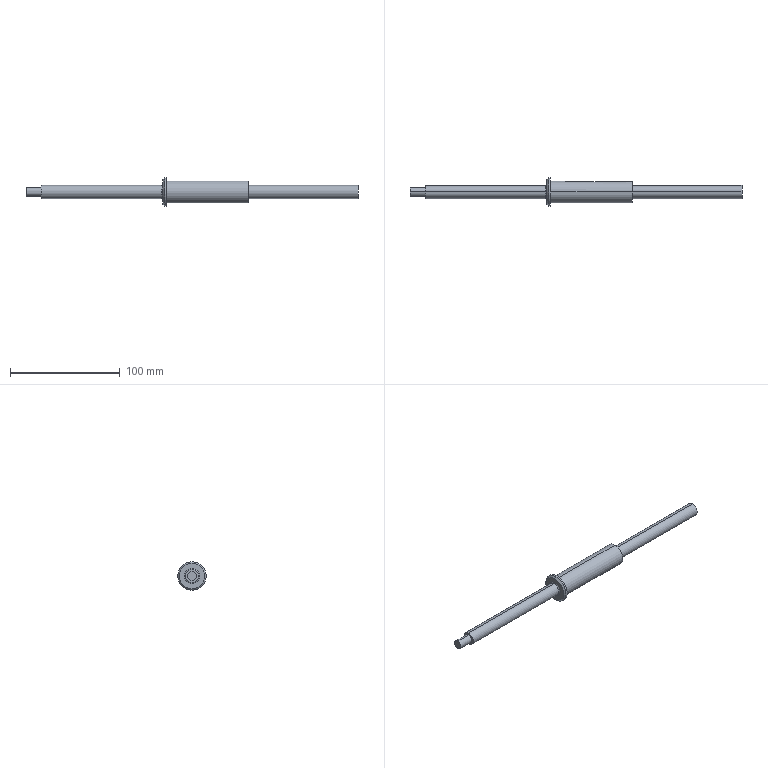Component | SolidWorks | ShortAxis(Modified)-1 | 1 solid | 28 faces | box 303 x 26 x 26 mm | volume 48394 mm3 | cylinder 11 | plane 9 | torus 6 | cone 2 | commonest cylinder face diameters 12 x4 8 x2 26 x2 20 x2 6 x1 | material AISI 1045 Steel, Cold Drawn
build123d program:
from build123d import *

# Parameters (mm, degrees)
FILLET3_R          = 0.5
FILLET6_R          = 1
CHAMFER1_SIZE      = 1.5
CUT_EXTRUDE1_DEPTH = 10


with BuildPart() as part:
    # Sketch1 → Revolve1 (revolve)
    with BuildSketch(Plane.XY, mode=Mode.PRIVATE) as revolve1_sk:
        Polygon((-152.849, 0), (-152.849, 6), (-52.849, 6), (-52.849, 10), (22.151, 10), (22.151, 13), (25.151, 13), (25.151, 6), (136.151, 6), (136.151, 4), (150.151, 4), (150.151, 0), align=None)
    revolve(revolve1_sk.sketch.rotate(Axis((-152.849, 0, 0), (1, 0, 0)), 90), axis=Axis((-152.849, 0, 0), (1, 0, 0)))

    # Fillet3
    fillet3_edges = [part.edges().sort_by_distance(p)[0] for p in [
        (22.151, 0, -10),
        (-52.849, 0, -6),
    ]]
    fillet(fillet3_edges, radius=FILLET3_R)

    # Fillet6
    fillet6_edges = [part.edges().sort_by_distance(p)[0] for p in [
        (25.151, 0, -6),
    ]]
    fillet(fillet6_edges, radius=FILLET6_R)

    # Chamfer1
    chamfer1_edges = [part.edges().sort_by_distance(p)[0] for p in [
        (25.151, 0, -13),
    ]]
    chamfer(chamfer1_edges, length=CHAMFER1_SIZE)

    # Sketch4 → Cut-Extrude1 (cut)
    with BuildSketch(Plane(origin=(0, 6.5, 0), x_dir=(1, 0, 0), z_dir=(0, 1, 0))):
        with BuildLine():
            Line((-63.443, -3), (7.151, -3))
            ThreePointArc((7.151, -3), (10.151, 0), (7.151, 3))
            Line((7.151, 3), (-63.443, 3))
            Line((-63.443, 3), (-63.443, -3))
        make_face()
    extrude(amount=CUT_EXTRUDE1_DEPTH, mode=Mode.SUBTRACT)


solid = part.part

# Placed as in the assembly
solid = solid.moved(Location((390.213, 15.116, 349), (-180, 0, 180)))
STEP:
#1=CARTESIAN_POINT('',(14.373,0.5951,14.193));
#2=VERTEX_POINT('',#1);
#3=CARTESIAN_POINT('',(14.373,0.5951,13.287));
#4=VERTEX_POINT('',#3);
#5=CARTESIAN_POINT('',(14.373,0.5951,13.74));
#6=DIRECTION('',(-1.,0.,0.));
#7=DIRECTION('',(0.,-0.,-1.));
#8=AXIS2_PLACEMENT_3D('',#5,#6,#7);
#9=CIRCLE('',#8,0.4528);
#10=EDGE_CURVE('',#2,#4,#9,.T.);
#11=ORIENTED_EDGE('',*,*,#10,.F.);
#12=CARTESIAN_POINT('',(14.432,0.5951,14.252));
#13=VERTEX_POINT('',#12);
#14=CARTESIAN_POINT('',(14.432,0.5951,14.252));
#15=DIRECTION('',(0.7071,0.,0.7071));
#16=VECTOR('',#15,39.37);
#17=LINE('',#14,#16);
#18=EDGE_CURVE('',#2,#13,#17,.T.);
#19=ORIENTED_EDGE('',*,*,#18,.T.);
#20=CARTESIAN_POINT('',(14.432,0.5951,13.228));
#21=VERTEX_POINT('',#20);
#22=CARTESIAN_POINT('',(14.432,0.5951,13.74));
#23=DIRECTION('',(1.,0.,0.));
#24=DIRECTION('',(0.,-0.,-1.));
#25=AXIS2_PLACEMENT_3D('',#22,#23,#24);
#26=CIRCLE('',#25,0.5118);
#27=EDGE_CURVE('',#21,#13,#26,.T.);
#28=ORIENTED_EDGE('',*,*,#27,.F.);
#29=CARTESIAN_POINT('',(14.432,0.5951,13.228));
#30=DIRECTION('',(0.7071,-0.,-0.7071));
#31=VECTOR('',#30,39.37);
#32=LINE('',#29,#31);
#33=EDGE_CURVE('',#4,#21,#32,.T.);
#34=ORIENTED_EDGE('',*,*,#33,.F.);
#35=EDGE_LOOP('',(#11,#19,#28,#34));
#36=FACE_OUTER_BOUND('',#35,.T.);
#37=CARTESIAN_POINT('',(14.432,0.5951,13.74));
#38=DIRECTION('',(1.,0.,0.));
#39=DIRECTION('',(0.,-0.,-1.));
#40=AXIS2_PLACEMENT_3D('',#37,#38,#39);
#41=CONICAL_SURFACE('',#40,0.5118,0.7854);
#42=ADVANCED_FACE('',(#36),#41,.T.);
#43=CARTESIAN_POINT('',(14.373,0.5951,14.016));
#44=VERTEX_POINT('',#43);
#45=CARTESIAN_POINT('',(14.373,0.5951,13.465));
#46=VERTEX_POINT('',#45);
#47=CARTESIAN_POINT('',(14.373,0.5951,13.74));
#48=DIRECTION('',(1.,0.,0.));
#49=DIRECTION('',(0.,0.,-1.));
#50=AXIS2_PLACEMENT_3D('',#47,#48,#49);
#51=CIRCLE('',#50,0.2756);
#52=EDGE_CURVE('',#44,#46,#51,.T.);
#53=ORIENTED_EDGE('',*,*,#52,.F.);
#54=CARTESIAN_POINT('',(14.333,0.5951,13.976));
#55=VERTEX_POINT('',#54);
#56=CARTESIAN_POINT('',(14.333,0.5951,14.016));
#57=DIRECTION('',(0.,1.,-0.));
#58=DIRECTION('',(0.,0.,1.));
#59=AXIS2_PLACEMENT_3D('',#56,#57,#58);
#60=CIRCLE('',#59,0.03937);
#61=EDGE_CURVE('',#44,#55,#60,.T.);
#62=ORIENTED_EDGE('',*,*,#61,.T.);
#63=CARTESIAN_POINT('',(14.333,0.5951,13.504));
#64=VERTEX_POINT('',#63);
#65=CARTESIAN_POINT('',(14.333,0.5951,13.74));
#66=DIRECTION('',(-1.,0.,0.));
#67=DIRECTION('',(0.,0.,-1.));
#68=AXIS2_PLACEMENT_3D('',#65,#66,#67);
#69=CIRCLE('',#68,0.2362);
#70=EDGE_CURVE('',#64,#55,#69,.T.);
#71=ORIENTED_EDGE('',*,*,#70,.F.);
#72=CARTESIAN_POINT('',(14.333,0.5951,13.465));
#73=DIRECTION('',(0.,-1.,0.));
#74=DIRECTION('',(0.,0.,-1.));
#75=AXIS2_PLACEMENT_3D('',#72,#73,#74);
#76=CIRCLE('',#75,0.03937);
#77=EDGE_CURVE('',#46,#64,#76,.T.);
#78=ORIENTED_EDGE('',*,*,#77,.F.);
#79=EDGE_LOOP('',(#53,#62,#71,#78));
#80=FACE_OUTER_BOUND('',#79,.T.);
#81=CARTESIAN_POINT('',(14.333,0.5951,13.74));
#82=DIRECTION('',(1.,0.,0.));
#83=DIRECTION('',(0.,-0.,-1.));
#84=AXIS2_PLACEMENT_3D('',#81,#82,#83);
#85=TOROIDAL_SURFACE('',#84,0.2756,0.03937);
#86=ADVANCED_FACE('',(#80),#85,.F.);
#87=CARTESIAN_POINT('',(17.443,0.5951,13.484));
#88=VERTEX_POINT('',#87);
#89=CARTESIAN_POINT('',(17.443,0.5951,13.996));
#90=VERTEX_POINT('',#89);
#91=CARTESIAN_POINT('',(17.443,0.5951,13.74));
#92=DIRECTION('',(-1.,0.,0.));
#93=DIRECTION('',(0.,0.,1.));
#94=AXIS2_PLACEMENT_3D('',#91,#92,#93);
#95=CIRCLE('',#94,0.2559);
#96=EDGE_CURVE('',#88,#90,#95,.T.);
#97=ORIENTED_EDGE('',*,*,#96,.F.);
#98=CARTESIAN_POINT('',(17.463,0.5951,13.504));
#99=VERTEX_POINT('',#98);
#100=CARTESIAN_POINT('',(17.463,0.5951,13.484));
#101=DIRECTION('',(0.,1.,0.));
#102=DIRECTION('',(0.,0.,1.));
#103=AXIS2_PLACEMENT_3D('',#100,#101,#102);
#104=CIRCLE('',#103,0.01969);
#105=EDGE_CURVE('',#88,#99,#104,.T.);
#106=ORIENTED_EDGE('',*,*,#105,.T.);
#107=CARTESIAN_POINT('',(17.463,0.5951,13.976));
#108=VERTEX_POINT('',#107);
#109=CARTESIAN_POINT('',(17.463,0.5951,13.74));
#110=DIRECTION('',(1.,0.,0.));
#111=DIRECTION('',(0.,0.,1.));
#112=AXIS2_PLACEMENT_3D('',#109,#110,#111);
#113=CIRCLE('',#112,0.2362);
#114=EDGE_CURVE('',#108,#99,#113,.T.);
#115=ORIENTED_EDGE('',*,*,#114,.F.);
#116=CARTESIAN_POINT('',(17.463,0.5951,13.996));
#117=DIRECTION('',(0.,-1.,0.));
#118=DIRECTION('',(0.,0.,-1.));
#119=AXIS2_PLACEMENT_3D('',#116,#117,#118);
#120=CIRCLE('',#119,0.01969);
#121=EDGE_CURVE('',#90,#108,#120,.T.);
#122=ORIENTED_EDGE('',*,*,#121,.F.);
#123=EDGE_LOOP('',(#97,#106,#115,#122));
#124=FACE_OUTER_BOUND('',#123,.T.);
#125=CARTESIAN_POINT('',(17.463,0.5951,13.74));
#126=DIRECTION('',(-1.,0.,0.));
#127=DIRECTION('',(0.,0.,1.));
#128=AXIS2_PLACEMENT_3D('',#125,#126,#127);
#129=TOROIDAL_SURFACE('',#128,0.2559,0.01969);
#130=ADVANCED_FACE('',(#124),#129,.F.);
#131=CARTESIAN_POINT('',(14.491,0.5951,13.327));
#132=VERTEX_POINT('',#131);
#133=CARTESIAN_POINT('',(14.491,0.5951,14.154));
#134=VERTEX_POINT('',#133);
#135=CARTESIAN_POINT('',(14.491,0.5951,13.74));
#136=DIRECTION('',(-1.,0.,0.));
#137=DIRECTION('',(0.,0.,1.));
#138=AXIS2_PLACEMENT_3D('',#135,#136,#137);
#139=CIRCLE('',#138,0.4134);
#140=EDGE_CURVE('',#132,#134,#139,.T.);
#141=ORIENTED_EDGE('',*,*,#140,.F.);
#142=CARTESIAN_POINT('',(14.51,0.5951,13.346));
#143=VERTEX_POINT('',#142);
#144=CARTESIAN_POINT('',(14.51,0.5951,13.327));
#145=DIRECTION('',(0.,1.,0.));
#146=DIRECTION('',(0.,0.,1.));
#147=AXIS2_PLACEMENT_3D('',#144,#145,#146);
#148=CIRCLE('',#147,0.01969);
#149=EDGE_CURVE('',#132,#143,#148,.T.);
#150=ORIENTED_EDGE('',*,*,#149,.T.);
#151=CARTESIAN_POINT('',(14.51,0.5951,14.134));
#152=VERTEX_POINT('',#151);
#153=CARTESIAN_POINT('',(14.51,0.5951,13.74));
#154=DIRECTION('',(1.,0.,0.));
#155=DIRECTION('',(0.,0.,1.));
#156=AXIS2_PLACEMENT_3D('',#153,#154,#155);
#157=CIRCLE('',#156,0.3937);
#158=EDGE_CURVE('',#152,#143,#157,.T.);
#159=ORIENTED_EDGE('',*,*,#158,.F.);
#160=CARTESIAN_POINT('',(14.51,0.5951,14.154));
#161=DIRECTION('',(0.,-1.,0.));
#162=DIRECTION('',(0.,0.,-1.));
#163=AXIS2_PLACEMENT_3D('',#160,#161,#162);
#164=CIRCLE('',#163,0.01969);
#165=EDGE_CURVE('',#134,#152,#164,.T.);
#166=ORIENTED_EDGE('',*,*,#165,.F.);
#167=EDGE_LOOP('',(#141,#150,#159,#166));
#168=FACE_OUTER_BOUND('',#167,.T.);
#169=CARTESIAN_POINT('',(14.51,0.5951,13.74));
#170=DIRECTION('',(-1.,0.,0.));
#171=DIRECTION('',(0.,0.,1.));
#172=AXIS2_PLACEMENT_3D('',#169,#170,#171);
#173=TOROIDAL_SURFACE('',#172,0.4134,0.01969);
#174=ADVANCED_FACE('',(#168),#173,.F.);
#175=CARTESIAN_POINT('',(9.451,0.5951,13.583));
#176=VERTEX_POINT('',#175);
#177=CARTESIAN_POINT('',(9.451,0.5951,13.898));
#178=VERTEX_POINT('',#177);
#179=CARTESIAN_POINT('',(9.451,0.5951,13.74));
#180=DIRECTION('',(1.,0.,0.));
#181=DIRECTION('',(0.,0.,-1.));
#182=AXIS2_PLACEMENT_3D('',#179,#180,#181);
#183=CIRCLE('',#182,0.1575);
#184=EDGE_CURVE('',#176,#178,#183,.T.);
#185=ORIENTED_EDGE('',*,*,#184,.T.);
#186=CARTESIAN_POINT('',(10.002,0.5951,13.898));
#187=VERTEX_POINT('',#186);
#188=CARTESIAN_POINT('',(21.38,0.5951,13.898));
#189=DIRECTION('',(1.,0.,0.));
#190=VECTOR('',#189,39.37);
#191=LINE('',#188,#190);
#192=EDGE_CURVE('',#178,#187,#191,.T.);
#193=ORIENTED_EDGE('',*,*,#192,.T.);
#194=CARTESIAN_POINT('',(10.002,0.5951,13.583));
#195=VERTEX_POINT('',#194);
#196=CARTESIAN_POINT('',(10.002,0.5951,13.74));
#197=DIRECTION('',(1.,0.,0.));
#198=DIRECTION('',(0.,0.,-1.));
#199=AXIS2_PLACEMENT_3D('',#196,#197,#198);
#200=CIRCLE('',#199,0.1575);
#201=EDGE_CURVE('',#195,#187,#200,.T.);
#202=ORIENTED_EDGE('',*,*,#201,.F.);
#203=CARTESIAN_POINT('',(21.38,0.5951,13.583));
#204=DIRECTION('',(1.,0.,0.));
#205=VECTOR('',#204,39.37);
#206=LINE('',#203,#205);
#207=EDGE_CURVE('',#176,#195,#206,.T.);
#208=ORIENTED_EDGE('',*,*,#207,.F.);
#209=EDGE_LOOP('',(#185,#193,#202,#208));
#210=FACE_OUTER_BOUND('',#209,.T.);
#211=CARTESIAN_POINT('',(21.38,0.5951,13.74));
#212=DIRECTION('',(1.,0.,0.));
#213=DIRECTION('',(0.,0.,-1.));
#214=AXIS2_PLACEMENT_3D('',#211,#212,#213);
#215=CYLINDRICAL_SURFACE('',#214,0.1575);
#216=ADVANCED_FACE('',(#210),#215,.T.);
#217=CARTESIAN_POINT('',(10.002,0.5951,13.504));
#218=VERTEX_POINT('',#217);
#219=CARTESIAN_POINT('',(10.002,0.5951,13.976));
#220=VERTEX_POINT('',#219);
#221=CARTESIAN_POINT('',(10.002,0.5951,13.74));
#222=DIRECTION('',(1.,0.,0.));
#223=DIRECTION('',(0.,0.,-1.));
#224=AXIS2_PLACEMENT_3D('',#221,#222,#223);
#225=CIRCLE('',#224,0.2362);
#226=EDGE_CURVE('',#218,#220,#225,.T.);
#227=ORIENTED_EDGE('',*,*,#226,.T.);
#228=CARTESIAN_POINT('',(21.38,0.5951,13.976));
#229=DIRECTION('',(1.,0.,0.));
#230=VECTOR('',#229,39.37);
#231=LINE('',#228,#230);
#232=EDGE_CURVE('',#220,#55,#231,.T.);
#233=ORIENTED_EDGE('',*,*,#232,.T.);
#234=CARTESIAN_POINT('',(14.333,0.5951,13.74));
#235=DIRECTION('',(-1.,0.,0.));
#236=DIRECTION('',(0.,0.,-1.));
#237=AXIS2_PLACEMENT_3D('',#234,#235,#236);
#238=CIRCLE('',#237,0.2362);
#239=EDGE_CURVE('',#55,#64,#238,.T.);
#240=ORIENTED_EDGE('',*,*,#239,.T.);
#241=CARTESIAN_POINT('',(21.38,0.5951,13.504));
#242=DIRECTION('',(1.,0.,0.));
#243=VECTOR('',#242,39.37);
#244=LINE('',#241,#243);
#245=EDGE_CURVE('',#218,#64,#244,.T.);
#246=ORIENTED_EDGE('',*,*,#245,.F.);
#247=EDGE_LOOP('',(#227,#233,#240,#246));
#248=FACE_OUTER_BOUND('',#247,.T.);
#249=CARTESIAN_POINT('',(21.38,0.5951,13.74));
#250=DIRECTION('',(1.,0.,0.));
#251=DIRECTION('',(0.,0.,-1.));
#252=AXIS2_PLACEMENT_3D('',#249,#250,#251);
#253=CYLINDRICAL_SURFACE('',#252,0.2362);
#254=ADVANCED_FACE('',(#248),#253,.T.);
#255=ORIENTED_EDGE('',*,*,#27,.T.);
#256=CARTESIAN_POINT('',(14.491,0.5951,14.252));
#257=VERTEX_POINT('',#256);
#258=CARTESIAN_POINT('',(21.38,0.5951,14.252));
#259=DIRECTION('',(1.,0.,0.));
#260=VECTOR('',#259,39.37);
#261=LINE('',#258,#260);
#262=EDGE_CURVE('',#13,#257,#261,.T.);
#263=ORIENTED_EDGE('',*,*,#262,.T.);
#264=CARTESIAN_POINT('',(14.491,0.5951,13.228));
#265=VERTEX_POINT('',#264);
#266=CARTESIAN_POINT('',(14.491,0.5951,13.74));
#267=DIRECTION('',(1.,0.,0.));
#268=DIRECTION('',(0.,-0.,-1.));
#269=AXIS2_PLACEMENT_3D('',#266,#267,#268);
#270=CIRCLE('',#269,0.5118);
#271=EDGE_CURVE('',#265,#257,#270,.T.);
#272=ORIENTED_EDGE('',*,*,#271,.F.);
#273=CARTESIAN_POINT('',(21.38,0.5951,13.228));
#274=DIRECTION('',(1.,0.,0.));
#275=VECTOR('',#274,39.37);
#276=LINE('',#273,#275);
#277=EDGE_CURVE('',#21,#265,#276,.T.);
#278=ORIENTED_EDGE('',*,*,#277,.F.);
#279=EDGE_LOOP('',(#255,#263,#272,#278));
#280=FACE_OUTER_BOUND('',#279,.T.);
#281=CARTESIAN_POINT('',(21.38,0.5951,13.74));
#282=DIRECTION('',(1.,0.,0.));
#283=DIRECTION('',(0.,-0.,-1.));
#284=AXIS2_PLACEMENT_3D('',#281,#282,#283);
#285=CYLINDRICAL_SURFACE('',#284,0.5118);
#286=ADVANCED_FACE('',(#280),#285,.T.);
#287=CARTESIAN_POINT('',(17.463,0.5951,13.74));
#288=DIRECTION('',(1.,0.,0.));
#289=DIRECTION('',(0.,0.,1.));
#290=AXIS2_PLACEMENT_3D('',#287,#288,#289);
#291=CIRCLE('',#290,0.2362);
#292=EDGE_CURVE('',#99,#108,#291,.T.);
#293=ORIENTED_EDGE('',*,*,#292,.T.);
#294=CARTESIAN_POINT('',(21.38,0.5951,13.976));
#295=VERTEX_POINT('',#294);
#296=CARTESIAN_POINT('',(21.38,0.5951,13.976));
#297=DIRECTION('',(1.,0.,0.));
#298=VECTOR('',#297,39.37);
#299=LINE('',#296,#298);
#300=EDGE_CURVE('',#108,#295,#299,.T.);
#301=ORIENTED_EDGE('',*,*,#300,.T.);
#302=CARTESIAN_POINT('',(21.38,0.5951,13.504));
#303=VERTEX_POINT('',#302);
#304=CARTESIAN_POINT('',(21.38,0.5951,13.74));
#305=DIRECTION('',(1.,0.,0.));
#306=DIRECTION('',(0.,0.,-1.));
#307=AXIS2_PLACEMENT_3D('',#304,#305,#306);
#308=CIRCLE('',#307,0.2362);
#309=EDGE_CURVE('',#303,#295,#308,.T.);
#310=ORIENTED_EDGE('',*,*,#309,.F.);
#311=CARTESIAN_POINT('',(21.38,0.5951,13.504));
#312=DIRECTION('',(1.,0.,0.));
#313=VECTOR('',#312,39.37);
#314=LINE('',#311,#313);
#315=EDGE_CURVE('',#99,#303,#314,.T.);
#316=ORIENTED_EDGE('',*,*,#315,.F.);
#317=EDGE_LOOP('',(#293,#301,#310,#316));
#318=FACE_OUTER_BOUND('',#317,.T.);
#319=CARTESIAN_POINT('',(21.38,0.5951,13.74));
#320=DIRECTION('',(1.,0.,0.));
#321=DIRECTION('',(0.,0.,-1.));
#322=AXIS2_PLACEMENT_3D('',#319,#320,#321);
#323=CYLINDRICAL_SURFACE('',#322,0.2362);
#324=ADVANCED_FACE('',(#318),#323,.T.);
#325=CARTESIAN_POINT('',(14.51,0.5951,13.74));
#326=DIRECTION('',(1.,0.,0.));
#327=DIRECTION('',(0.,0.,1.));
#328=AXIS2_PLACEMENT_3D('',#325,#326,#327);
#329=CIRCLE('',#328,0.3937);
#330=EDGE_CURVE('',#143,#152,#329,.T.);
#331=ORIENTED_EDGE('',*,*,#330,.T.);
#332=CARTESIAN_POINT('',(17.443,0.5951,14.134));
#333=VERTEX_POINT('',#332);
#334=CARTESIAN_POINT('',(21.38,0.5951,14.134));
#335=DIRECTION('',(1.,0.,0.));
#336=VECTOR('',#335,39.37);
#337=LINE('',#334,#336);
#338=EDGE_CURVE('',#152,#333,#337,.T.);
#339=ORIENTED_EDGE('',*,*,#338,.T.);
#340=CARTESIAN_POINT('',(17.443,0.9707,13.858));
#341=VERTEX_POINT('',#340);
#342=CARTESIAN_POINT('',(17.443,0.5951,13.74));
#343=DIRECTION('',(1.,0.,0.));
#344=DIRECTION('',(0.,-0.,-1.));
#345=AXIS2_PLACEMENT_3D('',#342,#343,#344);
#346=CIRCLE('',#345,0.3937);
#347=EDGE_CURVE('',#341,#333,#346,.T.);
#348=ORIENTED_EDGE('',*,*,#347,.F.);
#349=CARTESIAN_POINT('',(15.081,0.9707,13.858));
#350=VERTEX_POINT('',#349);
#351=CARTESIAN_POINT('',(21.38,0.9707,13.858));
#352=DIRECTION('',(1.,0.,0.));
#353=VECTOR('',#352,39.37);
#354=LINE('',#351,#353);
#355=EDGE_CURVE('',#350,#341,#354,.T.);
#356=ORIENTED_EDGE('',*,*,#355,.F.);
#357=CARTESIAN_POINT('',(15.081,0.9707,13.622));
#358=VERTEX_POINT('',#357);
#359=CARTESIAN_POINT('',(15.081,0.9707,13.622));
#360=CARTESIAN_POINT('',(15.073,0.9707,13.622));
#361=CARTESIAN_POINT('',(15.066,0.9709,13.623));
#362=CARTESIAN_POINT('',(15.05,0.9718,13.626));
#363=CARTESIAN_POINT('',(15.043,0.9725,13.628));
#364=CARTESIAN_POINT('',(15.029,0.9743,13.634));
#365=CARTESIAN_POINT('',(15.022,0.9753,13.638));
#366=CARTESIAN_POINT('',(15.009,0.9775,13.646));
#367=CARTESIAN_POINT('',(15.003,0.9787,13.651));
#368=CARTESIAN_POINT('',(14.987,0.9822,13.667));
#369=CARTESIAN_POINT('',(14.978,0.9845,13.681));
#370=CARTESIAN_POINT('',(14.969,0.987,13.702));
#371=CARTESIAN_POINT('',(14.967,0.9877,13.709));
#372=CARTESIAN_POINT('',(14.964,0.9886,13.725));
#373=CARTESIAN_POINT('',(14.963,0.9888,13.732));
#374=CARTESIAN_POINT('',(14.963,0.9888,13.748));
#375=CARTESIAN_POINT('',(14.964,0.9886,13.756));
#376=CARTESIAN_POINT('',(14.967,0.9877,13.771));
#377=CARTESIAN_POINT('',(14.969,0.987,13.778));
#378=CARTESIAN_POINT('',(14.975,0.9854,13.793));
#379=CARTESIAN_POINT('',(14.979,0.9844,13.799));
#380=CARTESIAN_POINT('',(14.987,0.9822,13.812));
#381=CARTESIAN_POINT('',(14.992,0.981,13.818));
#382=CARTESIAN_POINT('',(15.003,0.9787,13.829));
#383=CARTESIAN_POINT('',(15.009,0.9775,13.834));
#384=CARTESIAN_POINT('',(15.022,0.9753,13.843));
#385=CARTESIAN_POINT('',(15.029,0.9743,13.846));
#386=CARTESIAN_POINT('',(15.043,0.9726,13.852));
#387=CARTESIAN_POINT('',(15.05,0.9719,13.854));
#388=CARTESIAN_POINT('',(15.065,0.9709,13.857));
#389=CARTESIAN_POINT('',(15.073,0.9707,13.858));
#390=CARTESIAN_POINT('',(15.081,0.9707,13.858));
#391=B_SPLINE_CURVE_WITH_KNOTS('',3,(#359,#360,#361,#362,#363,#364,#365,#366,#367,#368,#369,#370,#371,#372,#373,#374,#375,#376,#377,#378,#379,#380,#381,#382,#383,#384,#385,#386,#387,#388,#389,#390),.UNSPECIFIED.,.F.,.F.,(4,2,2,2,2,2,2,2,2,2,2,2,2,2,2,4),(0.,0.0005894,0.001179,0.001768,0.002358,0.003536,0.004126,0.004715,0.005305,0.005894,0.006484,0.007073,0.007662,0.008252,0.008841,0.009431),.UNSPECIFIED.);
#392=EDGE_CURVE('',#358,#350,#391,.T.);
#393=ORIENTED_EDGE('',*,*,#392,.F.);
#394=CARTESIAN_POINT('',(17.443,0.9707,13.622));
#395=VERTEX_POINT('',#394);
#396=CARTESIAN_POINT('',(21.38,0.9707,13.622));
#397=DIRECTION('',(-1.,0.,0.));
#398=VECTOR('',#397,39.37);
#399=LINE('',#396,#398);
#400=EDGE_CURVE('',#395,#358,#399,.T.);
#401=ORIENTED_EDGE('',*,*,#400,.F.);
#402=CARTESIAN_POINT('',(17.443,0.5951,13.346));
#403=VERTEX_POINT('',#402);
#404=CARTESIAN_POINT('',(17.443,0.5951,13.74));
#405=DIRECTION('',(1.,0.,0.));
#406=DIRECTION('',(0.,-0.,-1.));
#407=AXIS2_PLACEMENT_3D('',#404,#405,#406);
#408=CIRCLE('',#407,0.3937);
#409=EDGE_CURVE('',#403,#395,#408,.T.);
#410=ORIENTED_EDGE('',*,*,#409,.F.);
#411=CARTESIAN_POINT('',(21.38,0.5951,13.346));
#412=DIRECTION('',(1.,0.,0.));
#413=VECTOR('',#412,39.37);
#414=LINE('',#411,#413);
#415=EDGE_CURVE('',#143,#403,#414,.T.);
#416=ORIENTED_EDGE('',*,*,#415,.F.);
#417=EDGE_LOOP('',(#331,#339,#348,#356,#393,#401,#410,#416));
#418=FACE_OUTER_BOUND('',#417,.T.);
#419=CARTESIAN_POINT('',(21.38,0.5951,13.74));
#420=DIRECTION('',(1.,0.,0.));
#421=DIRECTION('',(0.,-0.,-1.));
#422=AXIS2_PLACEMENT_3D('',#419,#420,#421);
#423=CYLINDRICAL_SURFACE('',#422,0.3937);
#424=ADVANCED_FACE('',(#418),#423,.T.);
#425=CARTESIAN_POINT('',(17.443,0.851,13.858));
#426=VERTEX_POINT('',#425);
#427=CARTESIAN_POINT('',(17.443,0.8313,13.858));
#428=DIRECTION('',(0.,-1.,0.));
#429=VECTOR('',#428,39.37);
#430=LINE('',#427,#429);
#431=EDGE_CURVE('',#341,#426,#430,.T.);
#432=ORIENTED_EDGE('',*,*,#431,.F.);
#433=ORIENTED_EDGE('',*,*,#347,.T.);
#434=CARTESIAN_POINT('',(17.443,0.5951,13.74));
#435=DIRECTION('',(1.,0.,0.));
#436=DIRECTION('',(0.,-0.,-1.));
#437=AXIS2_PLACEMENT_3D('',#434,#435,#436);
#438=CIRCLE('',#437,0.3937);
#439=EDGE_CURVE('',#333,#403,#438,.T.);
#440=ORIENTED_EDGE('',*,*,#439,.T.);
#441=ORIENTED_EDGE('',*,*,#409,.T.);
#442=CARTESIAN_POINT('',(17.443,0.851,13.622));
#443=VERTEX_POINT('',#442);
#444=CARTESIAN_POINT('',(17.443,0.8313,13.622));
#445=DIRECTION('',(0.,1.,-0.));
#446=VECTOR('',#445,39.37);
#447=LINE('',#444,#446);
#448=EDGE_CURVE('',#443,#395,#447,.T.);
#449=ORIENTED_EDGE('',*,*,#448,.F.);
#450=CARTESIAN_POINT('',(17.443,0.851,13.74));
#451=VERTEX_POINT('',#450);
#452=CARTESIAN_POINT('',(17.443,0.851,13.74));
#453=DIRECTION('',(0.,-0.,-1.));
#454=VECTOR('',#453,39.37);
#455=LINE('',#452,#454);
#456=EDGE_CURVE('',#451,#443,#455,.T.);
#457=ORIENTED_EDGE('',*,*,#456,.F.);
#458=CARTESIAN_POINT('',(17.443,0.5951,13.74));
#459=DIRECTION('',(-1.,0.,0.));
#460=DIRECTION('',(0.,0.,1.));
#461=AXIS2_PLACEMENT_3D('',#458,#459,#460);
#462=CIRCLE('',#461,0.2559);
#463=EDGE_CURVE('',#451,#88,#462,.T.);
#464=ORIENTED_EDGE('',*,*,#463,.T.);
#465=ORIENTED_EDGE('',*,*,#96,.T.);
#466=CARTESIAN_POINT('',(17.443,0.5951,13.74));
#467=DIRECTION('',(-1.,0.,0.));
#468=DIRECTION('',(0.,0.,1.));
#469=AXIS2_PLACEMENT_3D('',#466,#467,#468);
#470=CIRCLE('',#469,0.2559);
#471=EDGE_CURVE('',#90,#451,#470,.T.);
#472=ORIENTED_EDGE('',*,*,#471,.T.);
#473=CARTESIAN_POINT('',(17.443,0.851,13.74));
#474=DIRECTION('',(0.,-0.,-1.));
#475=VECTOR('',#474,39.37);
#476=LINE('',#473,#475);
#477=EDGE_CURVE('',#426,#451,#476,.T.);
#478=ORIENTED_EDGE('',*,*,#477,.F.);
#479=EDGE_LOOP('',(#432,#433,#440,#441,#449,#457,#464,#465,#472,#478));
#480=FACE_OUTER_BOUND('',#479,.T.);
#481=CARTESIAN_POINT('',(17.443,0.8313,13.74));
#482=DIRECTION('',(-1.,0.,0.));
#483=DIRECTION('',(0.,0.,1.));
#484=AXIS2_PLACEMENT_3D('',#481,#482,#483);
#485=PLANE('',#484);
#486=ADVANCED_FACE('',(#480),#485,.F.);
#487=ORIENTED_EDGE('',*,*,#338,.F.);
#488=ORIENTED_EDGE('',*,*,#158,.T.);
#489=ORIENTED_EDGE('',*,*,#415,.T.);
#490=ORIENTED_EDGE('',*,*,#439,.F.);
#491=EDGE_LOOP('',(#487,#488,#489,#490));
#492=FACE_OUTER_BOUND('',#491,.T.);
#493=CARTESIAN_POINT('',(21.38,0.5951,13.74));
#494=DIRECTION('',(1.,0.,0.));
#495=DIRECTION('',(0.,-0.,-1.));
#496=AXIS2_PLACEMENT_3D('',#493,#494,#495);
#497=CYLINDRICAL_SURFACE('',#496,0.3937);
#498=ADVANCED_FACE('',(#492),#497,.T.);
#499=ORIENTED_EDGE('',*,*,#309,.T.);
#500=CARTESIAN_POINT('',(21.38,0.5951,13.74));
#501=DIRECTION('',(1.,0.,0.));
#502=DIRECTION('',(0.,0.,-1.));
#503=AXIS2_PLACEMENT_3D('',#500,#501,#502);
#504=CIRCLE('',#503,0.2362);
#505=EDGE_CURVE('',#295,#303,#504,.T.);
#506=ORIENTED_EDGE('',*,*,#505,.T.);
#507=EDGE_LOOP('',(#499,#506));
#508=FACE_OUTER_BOUND('',#507,.T.);
#509=CARTESIAN_POINT('',(21.38,0.5951,13.74));
#510=DIRECTION('',(-1.,0.,0.));
#511=DIRECTION('',(0.,0.,1.));
#512=AXIS2_PLACEMENT_3D('',#509,#510,#511);
#513=PLANE('',#512);
#514=ADVANCED_FACE('',(#508),#513,.F.);
#515=ORIENTED_EDGE('',*,*,#300,.F.);
#516=ORIENTED_EDGE('',*,*,#114,.T.);
#517=ORIENTED_EDGE('',*,*,#315,.T.);
#518=ORIENTED_EDGE('',*,*,#505,.F.);
#519=EDGE_LOOP('',(#515,#516,#517,#518));
#520=FACE_OUTER_BOUND('',#519,.T.);
#521=CARTESIAN_POINT('',(21.38,0.5951,13.74));
#522=DIRECTION('',(1.,0.,0.));
#523=DIRECTION('',(0.,0.,-1.));
#524=AXIS2_PLACEMENT_3D('',#521,#522,#523);
#525=CYLINDRICAL_SURFACE('',#524,0.2362);
#526=ADVANCED_FACE('',(#520),#525,.T.);
#527=CARTESIAN_POINT('',(14.491,0.5951,13.74));
#528=DIRECTION('',(-1.,0.,0.));
#529=DIRECTION('',(0.,0.,1.));
#530=AXIS2_PLACEMENT_3D('',#527,#528,#529);
#531=CIRCLE('',#530,0.4134);
#532=EDGE_CURVE('',#134,#132,#531,.T.);
#533=ORIENTED_EDGE('',*,*,#532,.T.);
#534=ORIENTED_EDGE('',*,*,#140,.T.);
#535=EDGE_LOOP('',(#533,#534));
#536=FACE_BOUND('',#535,.T.);
#537=ORIENTED_EDGE('',*,*,#271,.T.);
#538=CARTESIAN_POINT('',(14.491,0.5951,13.74));
#539=DIRECTION('',(1.,0.,0.));
#540=DIRECTION('',(0.,-0.,-1.));
#541=AXIS2_PLACEMENT_3D('',#538,#539,#540);
#542=CIRCLE('',#541,0.5118);
#543=EDGE_CURVE('',#257,#265,#542,.T.);
#544=ORIENTED_EDGE('',*,*,#543,.T.);
#545=EDGE_LOOP('',(#537,#544));
#546=FACE_OUTER_BOUND('',#545,.T.);
#547=CARTESIAN_POINT('',(14.491,0.9888,13.74));
#548=DIRECTION('',(-1.,0.,0.));
#549=DIRECTION('',(0.,0.,1.));
#550=AXIS2_PLACEMENT_3D('',#547,#548,#549);
#551=PLANE('',#550);
#552=ADVANCED_FACE('',(#536,#546),#551,.F.);
#553=ORIENTED_EDGE('',*,*,#262,.F.);
#554=CARTESIAN_POINT('',(14.432,0.5951,13.74));
#555=DIRECTION('',(1.,0.,0.));
#556=DIRECTION('',(0.,-0.,-1.));
#557=AXIS2_PLACEMENT_3D('',#554,#555,#556);
#558=CIRCLE('',#557,0.5118);
#559=EDGE_CURVE('',#13,#21,#558,.T.);
#560=ORIENTED_EDGE('',*,*,#559,.T.);
#561=ORIENTED_EDGE('',*,*,#277,.T.);
#562=ORIENTED_EDGE('',*,*,#543,.F.);
#563=EDGE_LOOP('',(#553,#560,#561,#562));
#564=FACE_OUTER_BOUND('',#563,.T.);
#565=CARTESIAN_POINT('',(21.38,0.5951,13.74));
#566=DIRECTION('',(1.,0.,0.));
#567=DIRECTION('',(0.,-0.,-1.));
#568=AXIS2_PLACEMENT_3D('',#565,#566,#567);
#569=CYLINDRICAL_SURFACE('',#568,0.5118);
#570=ADVANCED_FACE('',(#564),#569,.T.);
#571=CARTESIAN_POINT('',(14.373,0.5951,13.74));
#572=DIRECTION('',(-1.,0.,0.));
#573=DIRECTION('',(0.,-0.,-1.));
#574=AXIS2_PLACEMENT_3D('',#571,#572,#573);
#575=CIRCLE('',#574,0.4528);
#576=EDGE_CURVE('',#4,#2,#575,.T.);
#577=ORIENTED_EDGE('',*,*,#576,.T.);
#578=ORIENTED_EDGE('',*,*,#10,.T.);
#579=EDGE_LOOP('',(#577,#578));
#580=FACE_OUTER_BOUND('',#579,.T.);
#581=CARTESIAN_POINT('',(14.373,0.5951,13.74));
#582=DIRECTION('',(1.,0.,0.));
#583=DIRECTION('',(0.,0.,-1.));
#584=AXIS2_PLACEMENT_3D('',#581,#582,#583);
#585=CIRCLE('',#584,0.2756);
#586=EDGE_CURVE('',#46,#44,#585,.T.);
#587=ORIENTED_EDGE('',*,*,#586,.T.);
#588=ORIENTED_EDGE('',*,*,#52,.T.);
#589=EDGE_LOOP('',(#587,#588));
#590=FACE_BOUND('',#589,.T.);
#591=CARTESIAN_POINT('',(14.373,1.107,13.74));
#592=DIRECTION('',(1.,0.,0.));
#593=DIRECTION('',(0.,-0.,-1.));
#594=AXIS2_PLACEMENT_3D('',#591,#592,#593);
#595=PLANE('',#594);
#596=ADVANCED_FACE('',(#580,#590),#595,.F.);
#597=ORIENTED_EDGE('',*,*,#232,.F.);
#598=CARTESIAN_POINT('',(10.002,0.5951,13.74));
#599=DIRECTION('',(1.,0.,0.));
#600=DIRECTION('',(0.,0.,-1.));
#601=AXIS2_PLACEMENT_3D('',#598,#599,#600);
#602=CIRCLE('',#601,0.2362);
#603=EDGE_CURVE('',#220,#218,#602,.T.);
#604=ORIENTED_EDGE('',*,*,#603,.T.);
#605=ORIENTED_EDGE('',*,*,#245,.T.);
#606=ORIENTED_EDGE('',*,*,#70,.T.);
#607=EDGE_LOOP('',(#597,#604,#605,#606));
#608=FACE_OUTER_BOUND('',#607,.T.);
#609=CARTESIAN_POINT('',(21.38,0.5951,13.74));
#610=DIRECTION('',(1.,0.,0.));
#611=DIRECTION('',(0.,0.,-1.));
#612=AXIS2_PLACEMENT_3D('',#609,#610,#611);
#613=CYLINDRICAL_SURFACE('',#612,0.2362);
#614=ADVANCED_FACE('',(#608),#613,.T.);
#615=ORIENTED_EDGE('',*,*,#226,.F.);
#616=ORIENTED_EDGE('',*,*,#603,.F.);
#617=EDGE_LOOP('',(#615,#616));
#618=FACE_OUTER_BOUND('',#617,.T.);
#619=ORIENTED_EDGE('',*,*,#201,.T.);
#620=CARTESIAN_POINT('',(10.002,0.5951,13.74));
#621=DIRECTION('',(1.,0.,0.));
#622=DIRECTION('',(0.,0.,-1.));
#623=AXIS2_PLACEMENT_3D('',#620,#621,#622);
#624=CIRCLE('',#623,0.1575);
#625=EDGE_CURVE('',#187,#195,#624,.T.);
#626=ORIENTED_EDGE('',*,*,#625,.T.);
#627=EDGE_LOOP('',(#619,#626));
#628=FACE_BOUND('',#627,.T.);
#629=CARTESIAN_POINT('',(10.002,0.8313,13.74));
#630=DIRECTION('',(1.,0.,0.));
#631=DIRECTION('',(0.,-0.,-1.));
#632=AXIS2_PLACEMENT_3D('',#629,#630,#631);
#633=PLANE('',#632);
#634=ADVANCED_FACE('',(#618,#628),#633,.F.);
#635=ORIENTED_EDGE('',*,*,#192,.F.);
#636=CARTESIAN_POINT('',(9.451,0.5951,13.74));
#637=DIRECTION('',(1.,0.,0.));
#638=DIRECTION('',(0.,0.,-1.));
#639=AXIS2_PLACEMENT_3D('',#636,#637,#638);
#640=CIRCLE('',#639,0.1575);
#641=EDGE_CURVE('',#178,#176,#640,.T.);
#642=ORIENTED_EDGE('',*,*,#641,.T.);
#643=ORIENTED_EDGE('',*,*,#207,.T.);
#644=ORIENTED_EDGE('',*,*,#625,.F.);
#645=EDGE_LOOP('',(#635,#642,#643,#644));
#646=FACE_OUTER_BOUND('',#645,.T.);
#647=CARTESIAN_POINT('',(21.38,0.5951,13.74));
#648=DIRECTION('',(1.,0.,0.));
#649=DIRECTION('',(0.,0.,-1.));
#650=AXIS2_PLACEMENT_3D('',#647,#648,#649);
#651=CYLINDRICAL_SURFACE('',#650,0.1575);
#652=ADVANCED_FACE('',(#646),#651,.T.);
#653=ORIENTED_EDGE('',*,*,#184,.F.);
#654=ORIENTED_EDGE('',*,*,#641,.F.);
#655=EDGE_LOOP('',(#653,#654));
#656=FACE_OUTER_BOUND('',#655,.T.);
#657=CARTESIAN_POINT('',(9.451,0.7526,13.74));
#658=DIRECTION('',(1.,0.,0.));
#659=DIRECTION('',(0.,-0.,-1.));
#660=AXIS2_PLACEMENT_3D('',#657,#658,#659);
#661=PLANE('',#660);
#662=ADVANCED_FACE('',(#656),#661,.F.);
#663=ORIENTED_EDGE('',*,*,#149,.F.);
#664=ORIENTED_EDGE('',*,*,#532,.F.);
#665=ORIENTED_EDGE('',*,*,#165,.T.);
#666=ORIENTED_EDGE('',*,*,#330,.F.);
#667=EDGE_LOOP('',(#663,#664,#665,#666));
#668=FACE_OUTER_BOUND('',#667,.T.);
#669=CARTESIAN_POINT('',(14.51,0.5951,13.74));
#670=DIRECTION('',(-1.,0.,0.));
#671=DIRECTION('',(0.,0.,1.));
#672=AXIS2_PLACEMENT_3D('',#669,#670,#671);
#673=TOROIDAL_SURFACE('',#672,0.4134,0.01969);
#674=ADVANCED_FACE('',(#668),#673,.F.);
#675=ORIENTED_EDGE('',*,*,#105,.F.);
#676=ORIENTED_EDGE('',*,*,#463,.F.);
#677=ORIENTED_EDGE('',*,*,#471,.F.);
#678=ORIENTED_EDGE('',*,*,#121,.T.);
#679=ORIENTED_EDGE('',*,*,#292,.F.);
#680=EDGE_LOOP('',(#675,#676,#677,#678,#679));
#681=FACE_OUTER_BOUND('',#680,.T.);
#682=CARTESIAN_POINT('',(17.463,0.5951,13.74));
#683=DIRECTION('',(-1.,0.,0.));
#684=DIRECTION('',(0.,0.,1.));
#685=AXIS2_PLACEMENT_3D('',#682,#683,#684);
#686=TOROIDAL_SURFACE('',#685,0.2559,0.01969);
#687=ADVANCED_FACE('',(#681),#686,.F.);
#688=ORIENTED_EDGE('',*,*,#61,.F.);
#689=ORIENTED_EDGE('',*,*,#586,.F.);
#690=ORIENTED_EDGE('',*,*,#77,.T.);
#691=ORIENTED_EDGE('',*,*,#239,.F.);
#692=EDGE_LOOP('',(#688,#689,#690,#691));
#693=FACE_OUTER_BOUND('',#692,.T.);
#694=CARTESIAN_POINT('',(14.333,0.5951,13.74));
#695=DIRECTION('',(1.,0.,0.));
#696=DIRECTION('',(0.,-0.,-1.));
#697=AXIS2_PLACEMENT_3D('',#694,#695,#696);
#698=TOROIDAL_SURFACE('',#697,0.2756,0.03937);
#699=ADVANCED_FACE('',(#693),#698,.F.);
#700=ORIENTED_EDGE('',*,*,#18,.F.);
#701=ORIENTED_EDGE('',*,*,#576,.F.);
#702=ORIENTED_EDGE('',*,*,#33,.T.);
#703=ORIENTED_EDGE('',*,*,#559,.F.);
#704=EDGE_LOOP('',(#700,#701,#702,#703));
#705=FACE_OUTER_BOUND('',#704,.T.);
#706=CARTESIAN_POINT('',(14.432,0.5951,13.74));
#707=DIRECTION('',(1.,0.,0.));
#708=DIRECTION('',(0.,-0.,-1.));
#709=AXIS2_PLACEMENT_3D('',#706,#707,#708);
#710=CONICAL_SURFACE('',#709,0.5118,0.7854);
#711=ADVANCED_FACE('',(#705),#710,.T.);
#712=ORIENTED_EDGE('',*,*,#392,.T.);
#713=CARTESIAN_POINT('',(15.081,0.851,13.858));
#714=VERTEX_POINT('',#713);
#715=CARTESIAN_POINT('',(15.081,1.245,13.858));
#716=DIRECTION('',(0.,-1.,0.));
#717=VECTOR('',#716,39.37);
#718=LINE('',#715,#717);
#719=EDGE_CURVE('',#350,#714,#718,.T.);
#720=ORIENTED_EDGE('',*,*,#719,.T.);
#721=CARTESIAN_POINT('',(15.081,0.851,13.622));
#722=VERTEX_POINT('',#721);
#723=CARTESIAN_POINT('',(15.081,0.851,13.74));
#724=DIRECTION('',(0.,1.,-0.));
#725=DIRECTION('',(0.,0.,-1.));
#726=AXIS2_PLACEMENT_3D('',#723,#724,#725);
#727=CIRCLE('',#726,0.1181);
#728=EDGE_CURVE('',#722,#714,#727,.T.);
#729=ORIENTED_EDGE('',*,*,#728,.F.);
#730=CARTESIAN_POINT('',(15.081,1.245,13.622));
#731=DIRECTION('',(0.,-1.,0.));
#732=VECTOR('',#731,39.37);
#733=LINE('',#730,#732);
#734=EDGE_CURVE('',#358,#722,#733,.T.);
#735=ORIENTED_EDGE('',*,*,#734,.F.);
#736=EDGE_LOOP('',(#712,#720,#729,#735));
#737=FACE_OUTER_BOUND('',#736,.T.);
#738=CARTESIAN_POINT('',(15.081,1.245,13.74));
#739=DIRECTION('',(0.,-1.,0.));
#740=DIRECTION('',(0.,0.,1.));
#741=AXIS2_PLACEMENT_3D('',#738,#739,#740);
#742=CYLINDRICAL_SURFACE('',#741,0.1181);
#743=ADVANCED_FACE('',(#737),#742,.F.);
#744=ORIENTED_EDGE('',*,*,#431,.T.);
#745=CARTESIAN_POINT('',(17.86,0.851,13.858));
#746=DIRECTION('',(1.,0.,0.));
#747=VECTOR('',#746,39.37);
#748=LINE('',#745,#747);
#749=EDGE_CURVE('',#714,#426,#748,.T.);
#750=ORIENTED_EDGE('',*,*,#749,.F.);
#751=ORIENTED_EDGE('',*,*,#719,.F.);
#752=ORIENTED_EDGE('',*,*,#355,.T.);
#753=EDGE_LOOP('',(#744,#750,#751,#752));
#754=FACE_OUTER_BOUND('',#753,.T.);
#755=CARTESIAN_POINT('',(17.86,1.245,13.858));
#756=DIRECTION('',(0.,-0.,-1.));
#757=DIRECTION('',(-1.,0.,0.));
#758=AXIS2_PLACEMENT_3D('',#755,#756,#757);
#759=PLANE('',#758);
#760=ADVANCED_FACE('',(#754),#759,.T.);
#761=ORIENTED_EDGE('',*,*,#448,.T.);
#762=ORIENTED_EDGE('',*,*,#400,.T.);
#763=ORIENTED_EDGE('',*,*,#734,.T.);
#764=CARTESIAN_POINT('',(17.86,0.851,13.622));
#765=DIRECTION('',(-1.,0.,0.));
#766=VECTOR('',#765,39.37);
#767=LINE('',#764,#766);
#768=EDGE_CURVE('',#443,#722,#767,.T.);
#769=ORIENTED_EDGE('',*,*,#768,.F.);
#770=EDGE_LOOP('',(#761,#762,#763,#769));
#771=FACE_OUTER_BOUND('',#770,.T.);
#772=CARTESIAN_POINT('',(17.86,1.245,13.622));
#773=DIRECTION('',(0.,0.,1.));
#774=DIRECTION('',(1.,0.,0.));
#775=AXIS2_PLACEMENT_3D('',#772,#773,#774);
#776=PLANE('',#775);
#777=ADVANCED_FACE('',(#771),#776,.T.);
#778=ORIENTED_EDGE('',*,*,#477,.T.);
#779=ORIENTED_EDGE('',*,*,#456,.T.);
#780=ORIENTED_EDGE('',*,*,#768,.T.);
#781=ORIENTED_EDGE('',*,*,#728,.T.);
#782=ORIENTED_EDGE('',*,*,#749,.T.);
#783=EDGE_LOOP('',(#778,#779,#780,#781,#782));
#784=FACE_OUTER_BOUND('',#783,.T.);
#785=CARTESIAN_POINT('',(15.081,0.851,13.74));
#786=DIRECTION('',(0.,1.,-0.));
#787=DIRECTION('',(0.,-0.,-1.));
#788=AXIS2_PLACEMENT_3D('',#785,#786,#787);
#789=PLANE('',#788);
#790=ADVANCED_FACE('',(#784),#789,.T.);
#791=CLOSED_SHELL('',(#42,#86,#130,#174,#216,#254,#286,#324,#424,#486,#498,#514,#526,#552,#570,#596,#614,#634,#652,#662,#674,#687,#699,#711,#743,#760,#777,#790));
#792=MANIFOLD_SOLID_BREP('',#791);
#793=CARTESIAN_POINT('',(0.,0.,0.));
#794=DIRECTION('',(0.,0.,1.));
#795=DIRECTION('',(1.,0.,0.));
#796=AXIS2_PLACEMENT_3D('',#793,#794,#795);
#797=(LENGTH_UNIT()NAMED_UNIT(*)SI_UNIT($,.METRE.));
#798=LENGTH_MEASURE_WITH_UNIT(LENGTH_MEASURE(0.0254),#797);
#799=DIMENSIONAL_EXPONENTS(1.,0.,0.,0.,0.,0.,0.);
#800=(CONVERSION_BASED_UNIT('',#798)LENGTH_UNIT()NAMED_UNIT(#799));
#801=UNCERTAINTY_MEASURE_WITH_UNIT(LENGTH_MEASURE(0.00001),#800,'','');
#802=(NAMED_UNIT(*)PLANE_ANGLE_UNIT()SI_UNIT($,.RADIAN.));
#803=(NAMED_UNIT(*)SI_UNIT($,.STERADIAN.)SOLID_ANGLE_UNIT());
#804=(GEOMETRIC_REPRESENTATION_CONTEXT(3)GLOBAL_UNCERTAINTY_ASSIGNED_CONTEXT((#801))GLOBAL_UNIT_ASSIGNED_CONTEXT((#800,#802,#803))REPRESENTATION_CONTEXT('',''));
#805=ADVANCED_BREP_SHAPE_REPRESENTATION('',(#792,#796),#804);
#806=COLOUR_RGB('',0.7922,0.8196,0.9333);
#807=FILL_AREA_STYLE_COLOUR('',#806);
#808=FILL_AREA_STYLE('',(#807));
#809=SURFACE_STYLE_FILL_AREA(#808);
#810=SURFACE_SIDE_STYLE('',(#809));
#811=SURFACE_STYLE_USAGE(.BOTH.,#810);
#812=PRESENTATION_STYLE_ASSIGNMENT((#811));
#813=STYLED_ITEM('',(#812),#792);
#814=PRESENTATION_LAYER_ASSIGNMENT('','',(#813));
#815=(LENGTH_UNIT()NAMED_UNIT(*)SI_UNIT($,.METRE.));
#816=LENGTH_MEASURE_WITH_UNIT(LENGTH_MEASURE(0.0254),#815);
#817=DIMENSIONAL_EXPONENTS(1.,0.,0.,0.,0.,0.,0.);
#818=(CONVERSION_BASED_UNIT('',#816)LENGTH_UNIT()NAMED_UNIT(#817));
#819=UNCERTAINTY_MEASURE_WITH_UNIT(LENGTH_MEASURE(0.00001),#818,'','');
#820=(NAMED_UNIT(*)PLANE_ANGLE_UNIT()SI_UNIT($,.RADIAN.));
#821=(NAMED_UNIT(*)SI_UNIT($,.STERADIAN.)SOLID_ANGLE_UNIT());
#822=(GEOMETRIC_REPRESENTATION_CONTEXT(3)GLOBAL_UNCERTAINTY_ASSIGNED_CONTEXT((#819))GLOBAL_UNIT_ASSIGNED_CONTEXT((#818,#820,#821))REPRESENTATION_CONTEXT('',''));
#823=MECHANICAL_DESIGN_GEOMETRIC_PRESENTATION_REPRESENTATION('',(#813),#822);